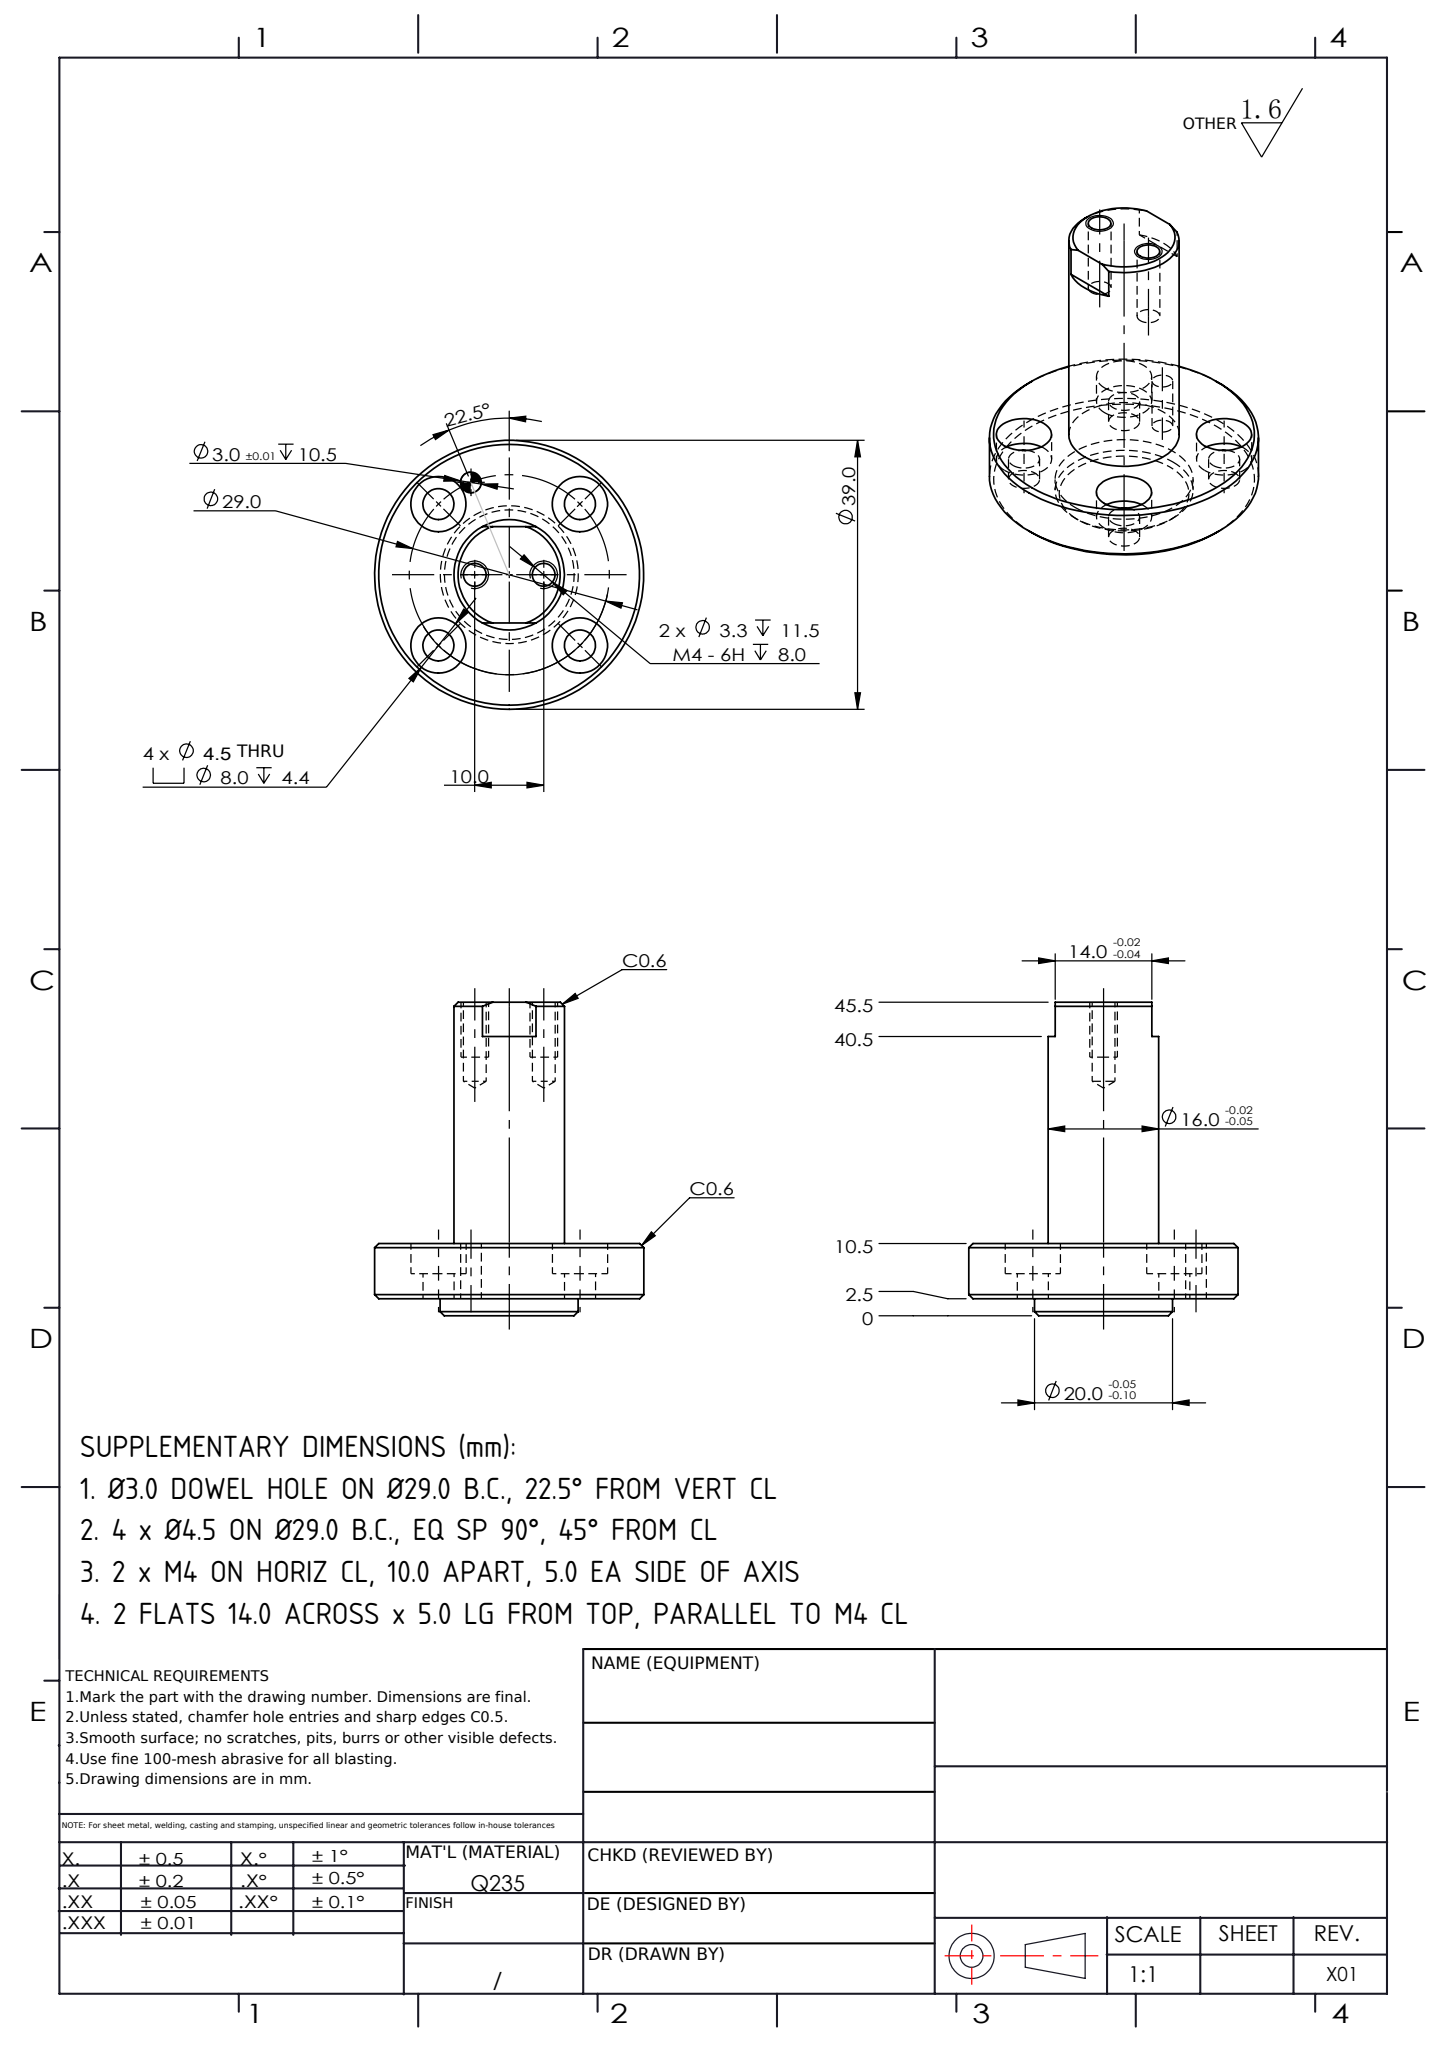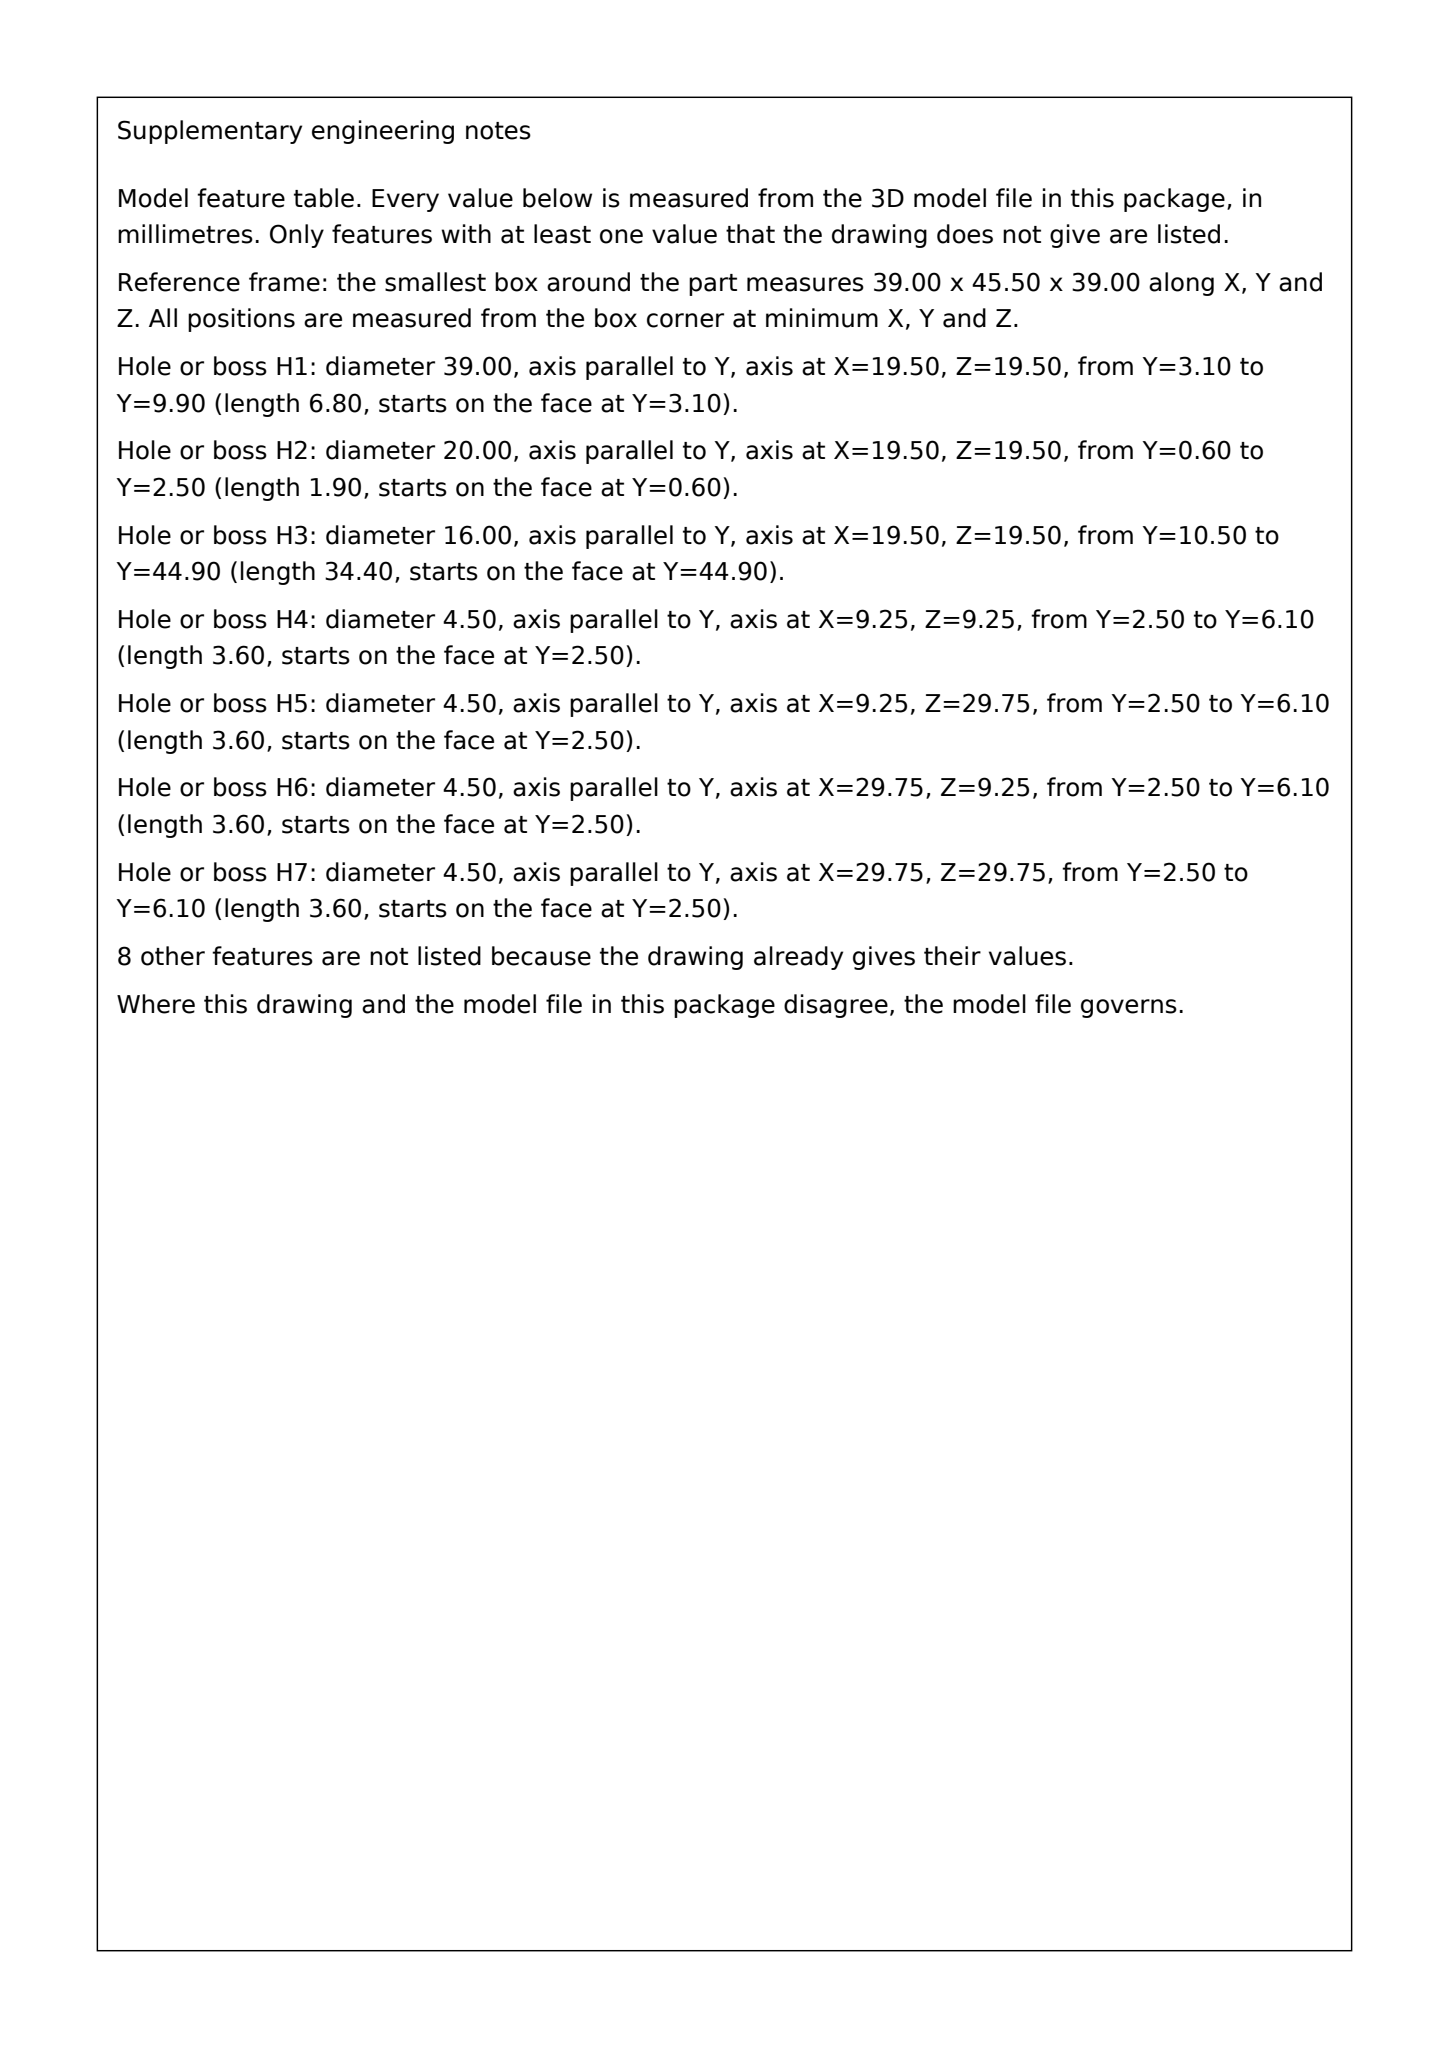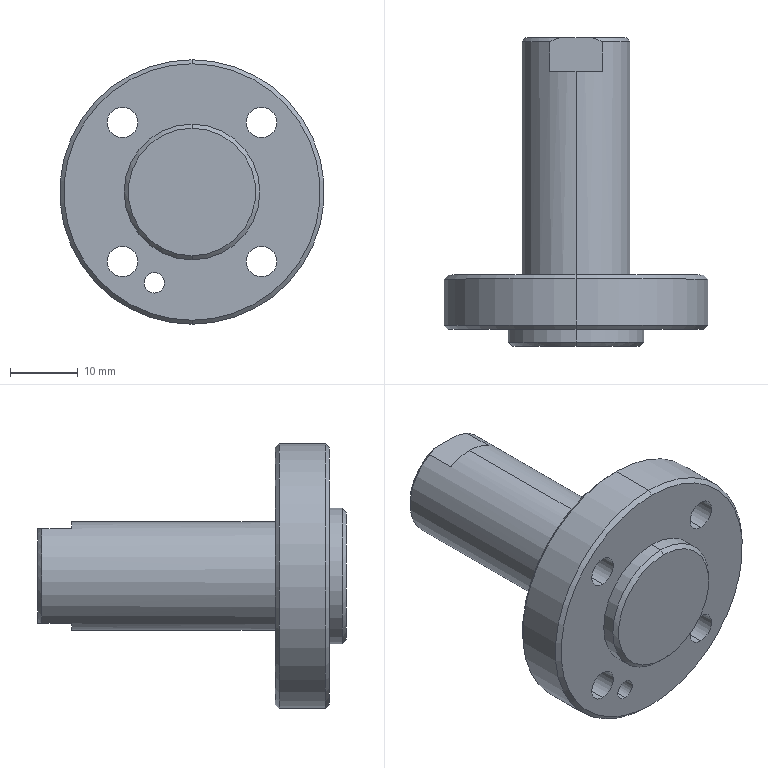Part | SolidWorks | mm | 1 solid | 52 faces | box 39 x 45.5 x 39 mm | volume 15893 mm3 | cylinder 28 | cone 12 | plane 12 | commonest cylinder face diameters 8 x8 4.5 x8 3.3 x4 3 x2 20 x2 39 x2 16 x2